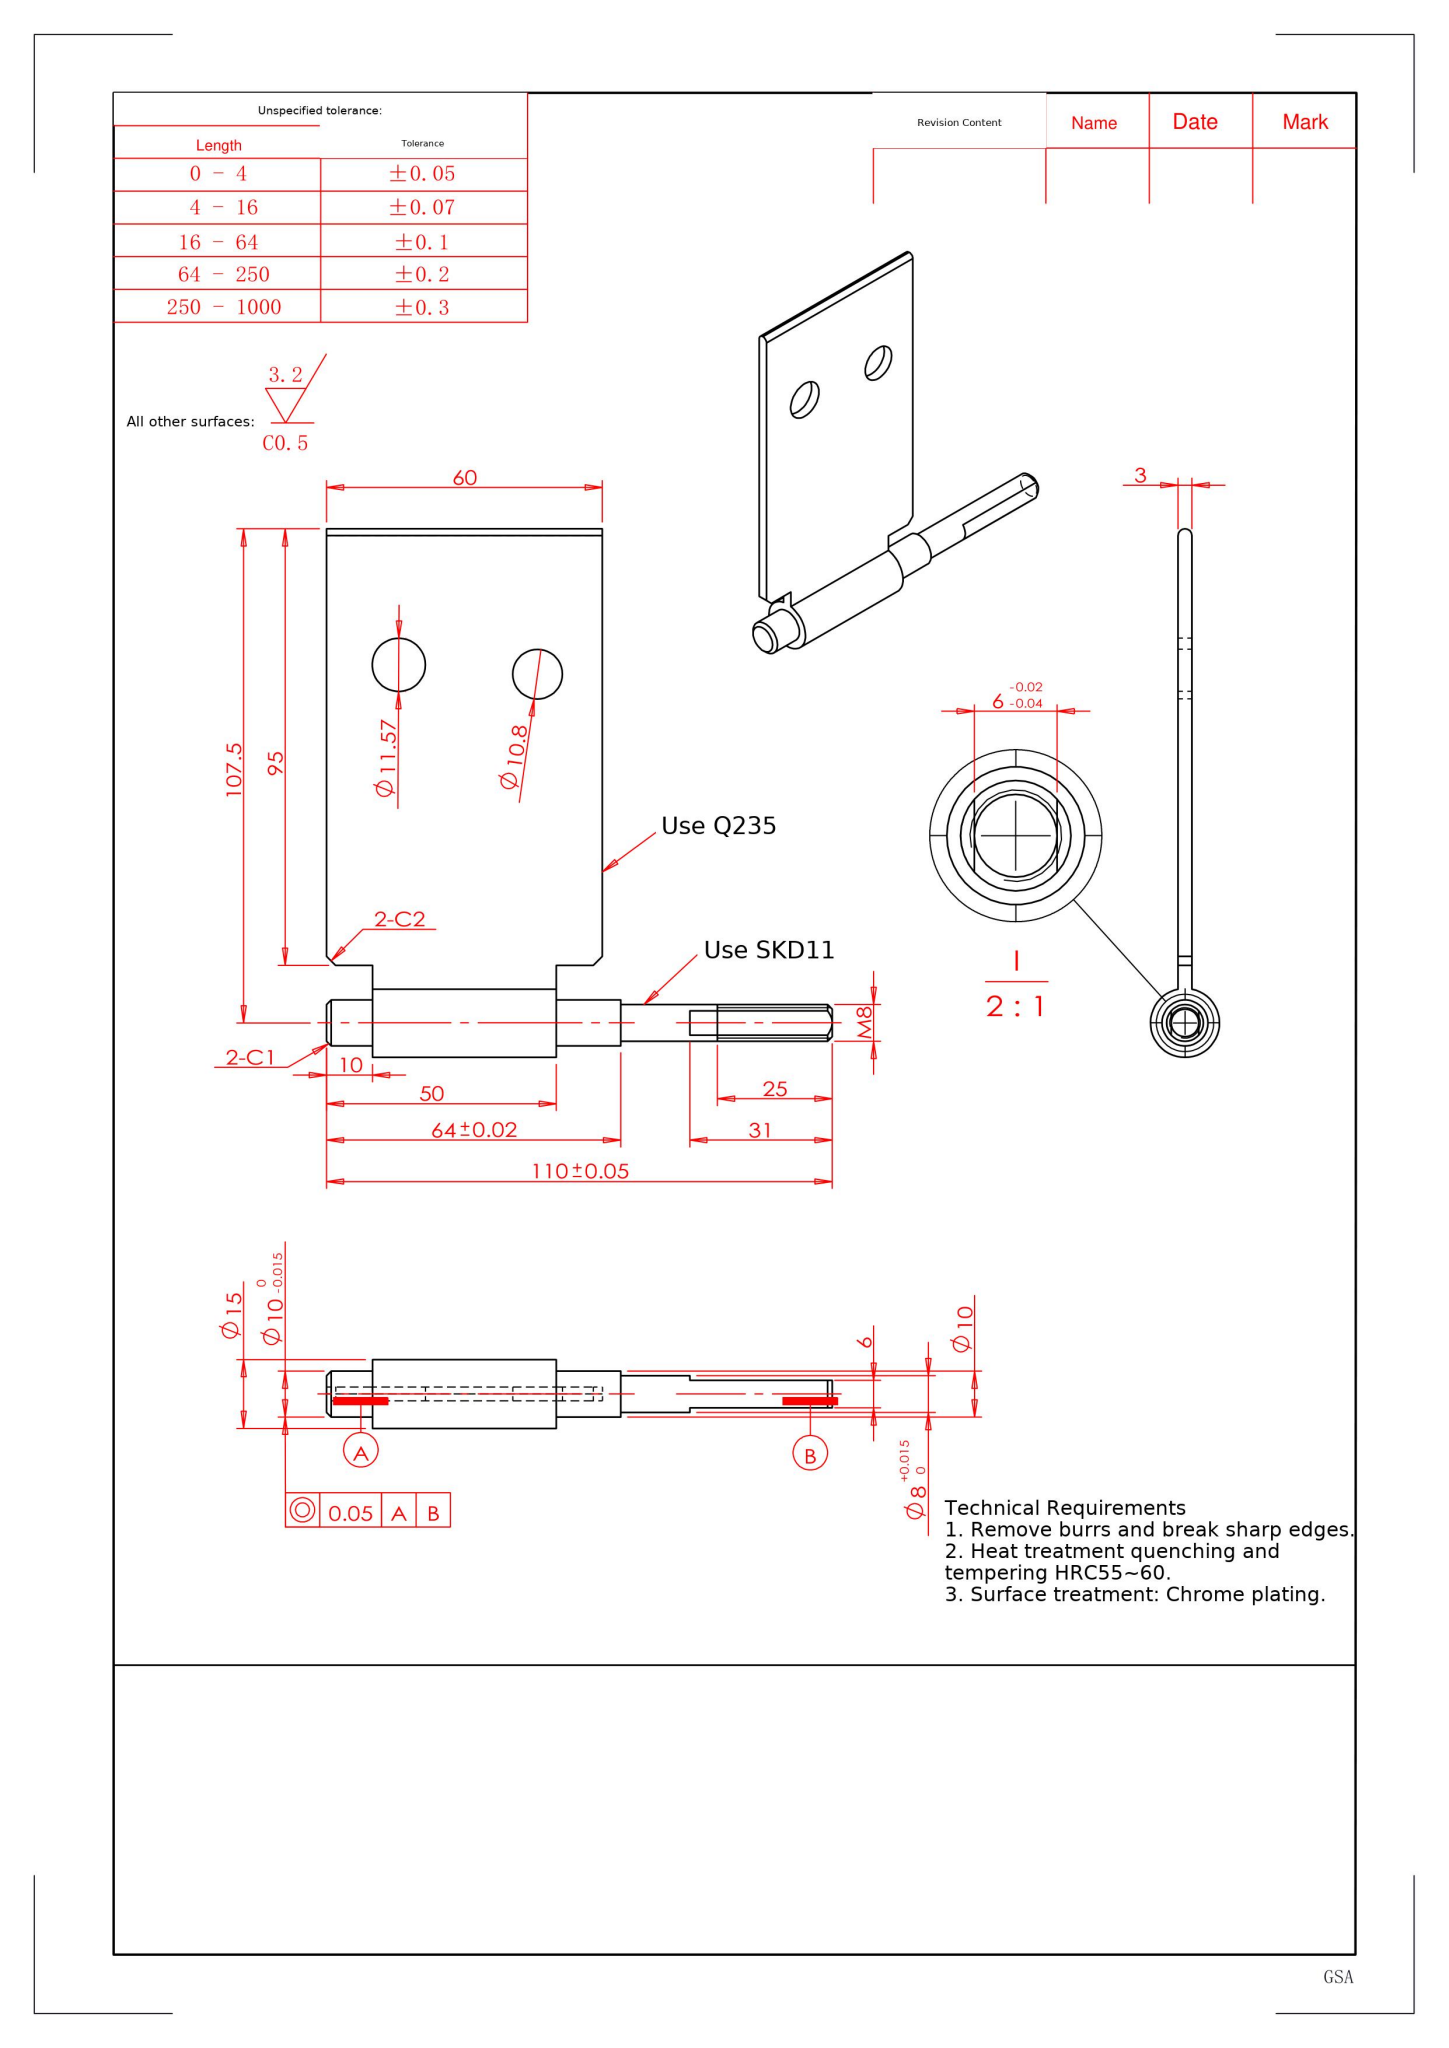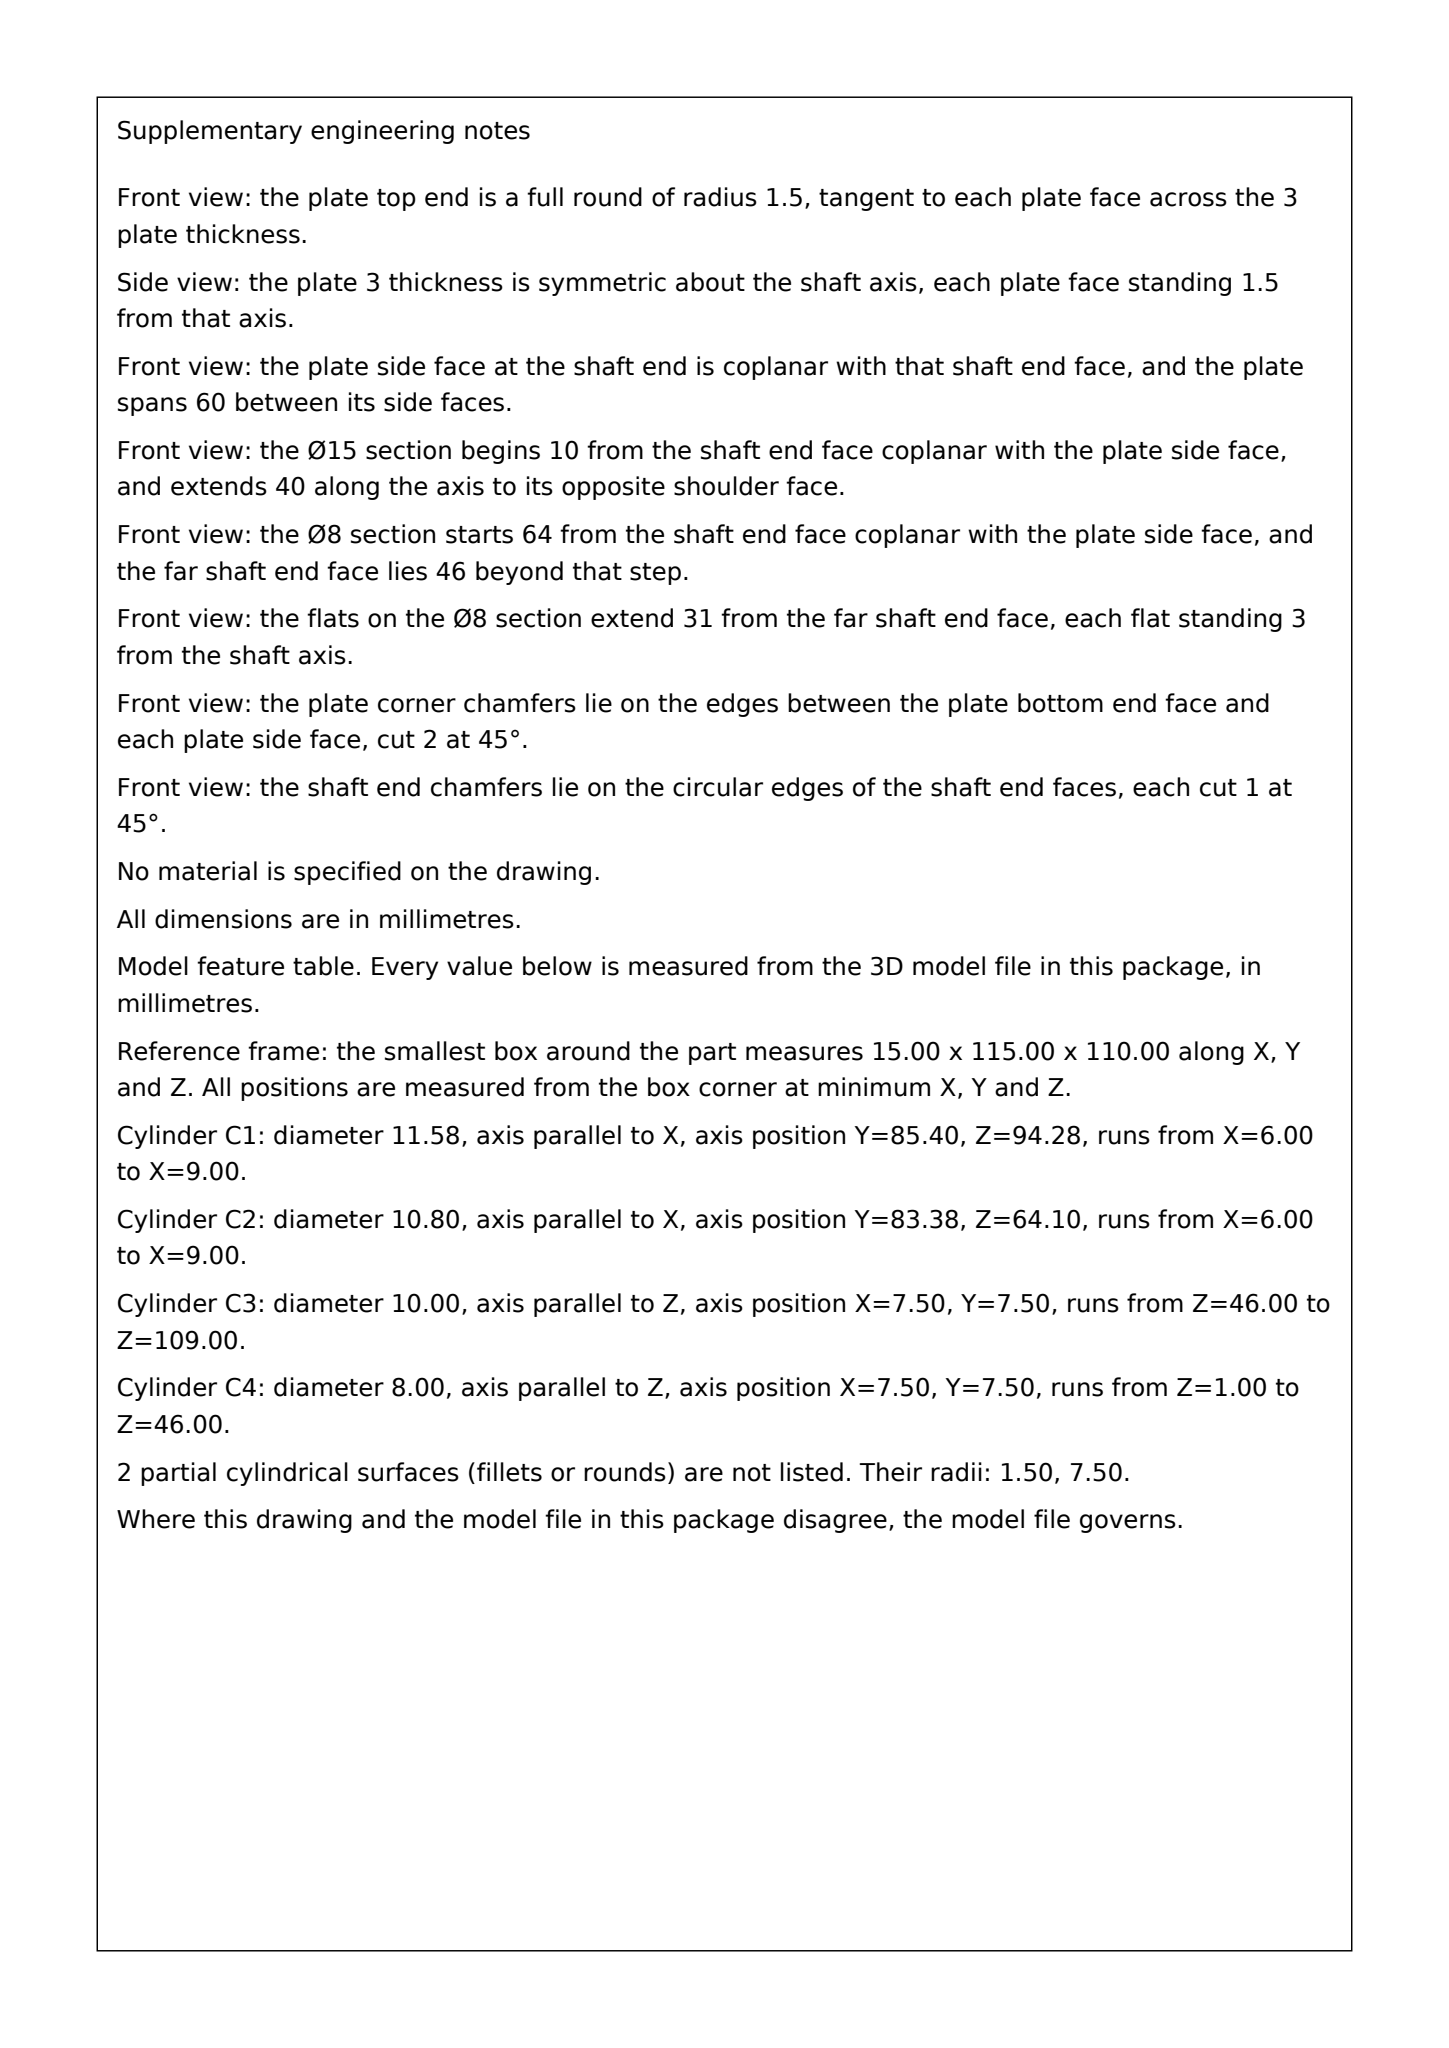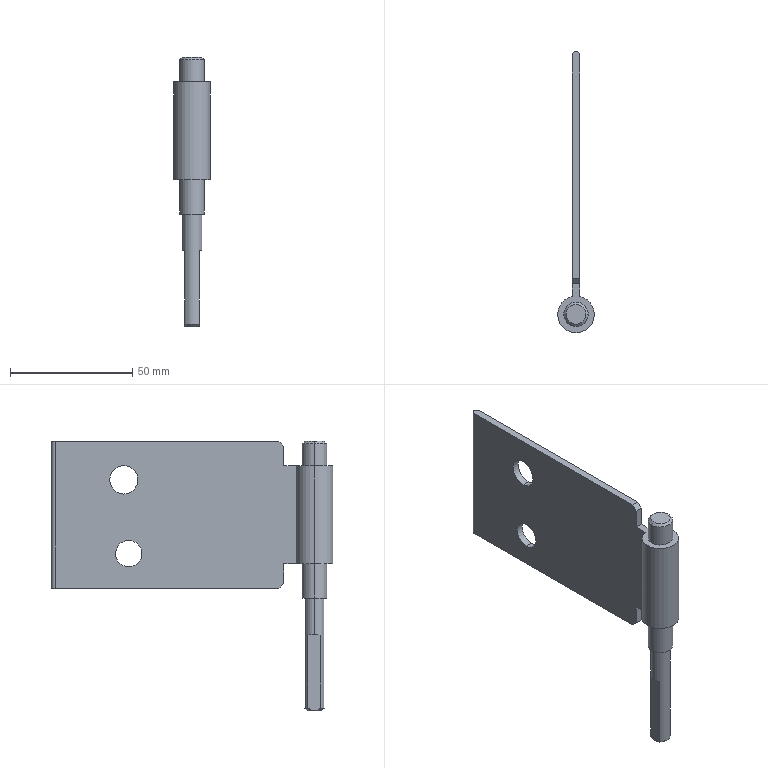Part | SolidWorks | mm | 1 solid | 36 faces | box 15 x 115 x 110 mm | volume 28065 mm3 | plane 17 | cylinder 15 | cone 4 | commonest cylinder face diameters 10 x4 15 x3 11.573 x2 10.804 x2 8 x2 3 x2